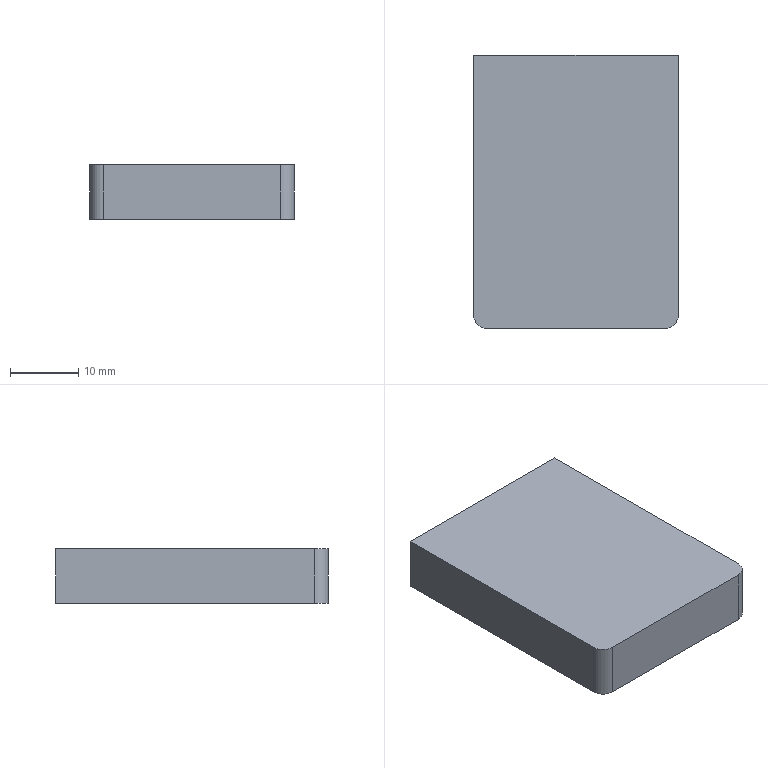Component | SolidWorks | GripperJaw2-1 | 1 solid | 8 faces | box 30 x 40 x 8 mm | volume 9586 mm3 | plane 6 | cylinder 2 | commonest cylinder face diameters 4 x2 | material 1060 Alloy
build123d program:
from build123d import *

# Parameters (mm, degrees)
SKETCH1_W           = 30
SKETCH1_H           = 40
BOSS_EXTRUDE1_DEPTH = 8
FILLET1_R           = 2


with BuildPart() as part:
    # Sketch1 → Boss-Extrude1 (new body)
    with BuildSketch(Plane.XY):
        Rectangle(SKETCH1_W, SKETCH1_H)
    extrude(amount=BOSS_EXTRUDE1_DEPTH)

    # Fillet1
    fillet1_edges = [part.edges().sort_by_distance(p)[0] for p in [
        (15, -20, 4),
        (-15, -20, 4),
    ]]
    fillet(fillet1_edges, radius=FILLET1_R)


solid = part.part

# Placed as in the assembly
solid = solid.moved(Location((-45.188, -89.343, 182.72), (0, 0, 0)))
STEP:
#1=COLOUR_RGB('',0.7922,0.8196,0.9333);
#2=FILL_AREA_STYLE_COLOUR('',#1);
#3=FILL_AREA_STYLE('',(#2));
#4=SURFACE_STYLE_FILL_AREA(#3);
#5=SURFACE_SIDE_STYLE('',(#4));
#6=SURFACE_STYLE_USAGE(.BOTH.,#5);
#7=PRESENTATION_STYLE_ASSIGNMENT((#6));
#8=CARTESIAN_POINT('',(-1.188,-4.226,7.509));
#9=VERTEX_POINT('',#8);
#10=CARTESIAN_POINT('',(-1.188,-2.73,7.509));
#11=VERTEX_POINT('',#10);
#12=CARTESIAN_POINT('',(-1.188,-2.73,7.509));
#13=DIRECTION('',(-0.,1.,0.));
#14=VECTOR('',#13,39.37);
#15=LINE('',#12,#14);
#16=EDGE_CURVE('',#9,#11,#15,.T.);
#17=ORIENTED_EDGE('',*,*,#16,.F.);
#18=CARTESIAN_POINT('',(-1.188,-4.226,7.194));
#19=VERTEX_POINT('',#18);
#20=CARTESIAN_POINT('',(-1.188,-4.226,7.509));
#21=DIRECTION('',(0.,0.,-1.));
#22=VECTOR('',#21,39.37);
#23=LINE('',#20,#22);
#24=EDGE_CURVE('',#9,#19,#23,.T.);
#25=ORIENTED_EDGE('',*,*,#24,.T.);
#26=CARTESIAN_POINT('',(-1.188,-2.73,7.194));
#27=VERTEX_POINT('',#26);
#28=CARTESIAN_POINT('',(-1.188,-2.73,7.194));
#29=DIRECTION('',(-0.,1.,0.));
#30=VECTOR('',#29,39.37);
#31=LINE('',#28,#30);
#32=EDGE_CURVE('',#19,#27,#31,.T.);
#33=ORIENTED_EDGE('',*,*,#32,.T.);
#34=CARTESIAN_POINT('',(-1.188,-2.73,7.509));
#35=DIRECTION('',(0.,0.,-1.));
#36=VECTOR('',#35,39.37);
#37=LINE('',#34,#36);
#38=EDGE_CURVE('',#11,#27,#37,.T.);
#39=ORIENTED_EDGE('',*,*,#38,.F.);
#40=EDGE_LOOP('',(#17,#25,#33,#39));
#41=FACE_OUTER_BOUND('',#40,.T.);
#42=CARTESIAN_POINT('',(-1.188,-2.73,7.509));
#43=DIRECTION('',(-1.,-0.,0.));
#44=DIRECTION('',(0.,-1.,0.));
#45=AXIS2_PLACEMENT_3D('',#42,#43,#44);
#46=PLANE('',#45);
#47=ADVANCED_FACE('',(#41),#46,.F.);
#48=CARTESIAN_POINT('',(-2.37,-2.73,7.194));
#49=VERTEX_POINT('',#48);
#50=CARTESIAN_POINT('',(-2.37,-2.73,7.194));
#51=DIRECTION('',(-1.,0.,0.));
#52=VECTOR('',#51,39.37);
#53=LINE('',#50,#52);
#54=EDGE_CURVE('',#27,#49,#53,.T.);
#55=ORIENTED_EDGE('',*,*,#54,.T.);
#56=CARTESIAN_POINT('',(-2.37,-2.73,7.509));
#57=VERTEX_POINT('',#56);
#58=CARTESIAN_POINT('',(-2.37,-2.73,7.509));
#59=DIRECTION('',(0.,0.,-1.));
#60=VECTOR('',#59,39.37);
#61=LINE('',#58,#60);
#62=EDGE_CURVE('',#57,#49,#61,.T.);
#63=ORIENTED_EDGE('',*,*,#62,.F.);
#64=CARTESIAN_POINT('',(-2.37,-2.73,7.509));
#65=DIRECTION('',(-1.,0.,0.));
#66=VECTOR('',#65,39.37);
#67=LINE('',#64,#66);
#68=EDGE_CURVE('',#11,#57,#67,.T.);
#69=ORIENTED_EDGE('',*,*,#68,.F.);
#70=ORIENTED_EDGE('',*,*,#38,.T.);
#71=EDGE_LOOP('',(#55,#63,#69,#70));
#72=FACE_OUTER_BOUND('',#71,.T.);
#73=CARTESIAN_POINT('',(-2.37,-2.73,7.509));
#74=DIRECTION('',(0.,-1.,0.));
#75=DIRECTION('',(0.,0.,-1.));
#76=AXIS2_PLACEMENT_3D('',#73,#74,#75);
#77=PLANE('',#76);
#78=ADVANCED_FACE('',(#72),#77,.F.);
#79=CARTESIAN_POINT('',(-2.37,-4.226,7.194));
#80=VERTEX_POINT('',#79);
#81=CARTESIAN_POINT('',(-2.37,-2.73,7.194));
#82=DIRECTION('',(0.,-1.,0.));
#83=VECTOR('',#82,39.37);
#84=LINE('',#81,#83);
#85=EDGE_CURVE('',#49,#80,#84,.T.);
#86=ORIENTED_EDGE('',*,*,#85,.T.);
#87=CARTESIAN_POINT('',(-2.37,-4.226,7.509));
#88=VERTEX_POINT('',#87);
#89=CARTESIAN_POINT('',(-2.37,-4.226,7.509));
#90=DIRECTION('',(0.,0.,1.));
#91=VECTOR('',#90,39.37);
#92=LINE('',#89,#91);
#93=EDGE_CURVE('',#80,#88,#92,.T.);
#94=ORIENTED_EDGE('',*,*,#93,.T.);
#95=CARTESIAN_POINT('',(-2.37,-2.73,7.509));
#96=DIRECTION('',(0.,-1.,0.));
#97=VECTOR('',#96,39.37);
#98=LINE('',#95,#97);
#99=EDGE_CURVE('',#57,#88,#98,.T.);
#100=ORIENTED_EDGE('',*,*,#99,.F.);
#101=ORIENTED_EDGE('',*,*,#62,.T.);
#102=EDGE_LOOP('',(#86,#94,#100,#101));
#103=FACE_OUTER_BOUND('',#102,.T.);
#104=CARTESIAN_POINT('',(-2.37,-2.73,7.509));
#105=DIRECTION('',(1.,0.,0.));
#106=DIRECTION('',(-0.,1.,0.));
#107=AXIS2_PLACEMENT_3D('',#104,#105,#106);
#108=PLANE('',#107);
#109=ADVANCED_FACE('',(#103),#108,.F.);
#110=CARTESIAN_POINT('',(-2.291,-4.305,7.194));
#111=VERTEX_POINT('',#110);
#112=CARTESIAN_POINT('',(-1.267,-4.305,7.194));
#113=VERTEX_POINT('',#112);
#114=CARTESIAN_POINT('',(-2.37,-4.305,7.194));
#115=DIRECTION('',(1.,0.,0.));
#116=VECTOR('',#115,39.37);
#117=LINE('',#114,#116);
#118=EDGE_CURVE('',#111,#113,#117,.T.);
#119=ORIENTED_EDGE('',*,*,#118,.T.);
#120=CARTESIAN_POINT('',(-1.267,-4.305,7.509));
#121=VERTEX_POINT('',#120);
#122=CARTESIAN_POINT('',(-1.267,-4.305,7.509));
#123=DIRECTION('',(0.,0.,1.));
#124=VECTOR('',#123,39.37);
#125=LINE('',#122,#124);
#126=EDGE_CURVE('',#113,#121,#125,.T.);
#127=ORIENTED_EDGE('',*,*,#126,.T.);
#128=CARTESIAN_POINT('',(-2.291,-4.305,7.509));
#129=VERTEX_POINT('',#128);
#130=CARTESIAN_POINT('',(-2.37,-4.305,7.509));
#131=DIRECTION('',(1.,0.,0.));
#132=VECTOR('',#131,39.37);
#133=LINE('',#130,#132);
#134=EDGE_CURVE('',#129,#121,#133,.T.);
#135=ORIENTED_EDGE('',*,*,#134,.F.);
#136=CARTESIAN_POINT('',(-2.291,-4.305,7.509));
#137=DIRECTION('',(0.,0.,-1.));
#138=VECTOR('',#137,39.37);
#139=LINE('',#136,#138);
#140=EDGE_CURVE('',#129,#111,#139,.T.);
#141=ORIENTED_EDGE('',*,*,#140,.T.);
#142=EDGE_LOOP('',(#119,#127,#135,#141));
#143=FACE_OUTER_BOUND('',#142,.T.);
#144=CARTESIAN_POINT('',(-2.37,-4.305,7.509));
#145=DIRECTION('',(0.,1.,0.));
#146=DIRECTION('',(0.,0.,1.));
#147=AXIS2_PLACEMENT_3D('',#144,#145,#146);
#148=PLANE('',#147);
#149=ADVANCED_FACE('',(#143),#148,.F.);
#150=ORIENTED_EDGE('',*,*,#134,.T.);
#151=CARTESIAN_POINT('',(-1.267,-4.226,7.509));
#152=DIRECTION('',(0.,0.,1.));
#153=DIRECTION('',(1.,0.,0.));
#154=AXIS2_PLACEMENT_3D('',#151,#152,#153);
#155=CIRCLE('',#154,0.07874);
#156=EDGE_CURVE('',#121,#9,#155,.T.);
#157=ORIENTED_EDGE('',*,*,#156,.T.);
#158=ORIENTED_EDGE('',*,*,#16,.T.);
#159=ORIENTED_EDGE('',*,*,#68,.T.);
#160=ORIENTED_EDGE('',*,*,#99,.T.);
#161=CARTESIAN_POINT('',(-2.291,-4.226,7.509));
#162=DIRECTION('',(0.,0.,1.));
#163=DIRECTION('',(1.,0.,0.));
#164=AXIS2_PLACEMENT_3D('',#161,#162,#163);
#165=CIRCLE('',#164,0.07874);
#166=EDGE_CURVE('',#88,#129,#165,.T.);
#167=ORIENTED_EDGE('',*,*,#166,.T.);
#168=EDGE_LOOP('',(#150,#157,#158,#159,#160,#167));
#169=FACE_OUTER_BOUND('',#168,.T.);
#170=CARTESIAN_POINT('',(-1.779,-3.517,7.509));
#171=DIRECTION('',(0.,0.,1.));
#172=DIRECTION('',(1.,0.,0.));
#173=AXIS2_PLACEMENT_3D('',#170,#171,#172);
#174=PLANE('',#173);
#175=ADVANCED_FACE('',(#169),#174,.T.);
#176=ORIENTED_EDGE('',*,*,#32,.F.);
#177=CARTESIAN_POINT('',(-1.267,-4.226,7.194));
#178=DIRECTION('',(0.,0.,-1.));
#179=DIRECTION('',(1.,0.,0.));
#180=AXIS2_PLACEMENT_3D('',#177,#178,#179);
#181=CIRCLE('',#180,0.07874);
#182=EDGE_CURVE('',#19,#113,#181,.T.);
#183=ORIENTED_EDGE('',*,*,#182,.T.);
#184=ORIENTED_EDGE('',*,*,#118,.F.);
#185=CARTESIAN_POINT('',(-2.291,-4.226,7.194));
#186=DIRECTION('',(0.,0.,-1.));
#187=DIRECTION('',(1.,0.,0.));
#188=AXIS2_PLACEMENT_3D('',#185,#186,#187);
#189=CIRCLE('',#188,0.07874);
#190=EDGE_CURVE('',#111,#80,#189,.T.);
#191=ORIENTED_EDGE('',*,*,#190,.T.);
#192=ORIENTED_EDGE('',*,*,#85,.F.);
#193=ORIENTED_EDGE('',*,*,#54,.F.);
#194=EDGE_LOOP('',(#176,#183,#184,#191,#192,#193));
#195=FACE_OUTER_BOUND('',#194,.T.);
#196=CARTESIAN_POINT('',(-1.779,-3.517,7.194));
#197=DIRECTION('',(0.,0.,1.));
#198=DIRECTION('',(1.,0.,0.));
#199=AXIS2_PLACEMENT_3D('',#196,#197,#198);
#200=PLANE('',#199);
#201=ADVANCED_FACE('',(#195),#200,.F.);
#202=ORIENTED_EDGE('',*,*,#156,.F.);
#203=ORIENTED_EDGE('',*,*,#126,.F.);
#204=ORIENTED_EDGE('',*,*,#182,.F.);
#205=ORIENTED_EDGE('',*,*,#24,.F.);
#206=EDGE_LOOP('',(#202,#203,#204,#205));
#207=FACE_OUTER_BOUND('',#206,.T.);
#208=CARTESIAN_POINT('',(-1.267,-4.226,7.509));
#209=DIRECTION('',(0.,0.,-1.));
#210=DIRECTION('',(-1.,0.,0.));
#211=AXIS2_PLACEMENT_3D('',#208,#209,#210);
#212=CYLINDRICAL_SURFACE('',#211,0.07874);
#213=ADVANCED_FACE('',(#207),#212,.T.);
#214=ORIENTED_EDGE('',*,*,#166,.F.);
#215=ORIENTED_EDGE('',*,*,#93,.F.);
#216=ORIENTED_EDGE('',*,*,#190,.F.);
#217=ORIENTED_EDGE('',*,*,#140,.F.);
#218=EDGE_LOOP('',(#214,#215,#216,#217));
#219=FACE_OUTER_BOUND('',#218,.T.);
#220=CARTESIAN_POINT('',(-2.291,-4.226,7.509));
#221=DIRECTION('',(0.,0.,-1.));
#222=DIRECTION('',(-1.,0.,0.));
#223=AXIS2_PLACEMENT_3D('',#220,#221,#222);
#224=CYLINDRICAL_SURFACE('',#223,0.07874);
#225=ADVANCED_FACE('',(#219),#224,.T.);
#226=CLOSED_SHELL('',(#47,#78,#109,#149,#175,#201,#213,#225));
#227=MANIFOLD_SOLID_BREP('',#226);
#228=STYLED_ITEM('',(#7),#227);
#229=PRESENTATION_LAYER_ASSIGNMENT('','',(#228));
#230=CARTESIAN_POINT('',(0.,0.,0.));
#231=DIRECTION('',(0.,0.,1.));
#232=DIRECTION('',(1.,0.,0.));
#233=AXIS2_PLACEMENT_3D('',#230,#231,#232);
#234=(LENGTH_UNIT()NAMED_UNIT(*)SI_UNIT($,.METRE.));
#235=LENGTH_MEASURE_WITH_UNIT(LENGTH_MEASURE(0.0254),#234);
#236=DIMENSIONAL_EXPONENTS(1.,0.,0.,0.,0.,0.,0.);
#237=(CONVERSION_BASED_UNIT('',#235)LENGTH_UNIT()NAMED_UNIT(#236));
#238=UNCERTAINTY_MEASURE_WITH_UNIT(LENGTH_MEASURE(0.00001),#237,'','');
#239=(NAMED_UNIT(*)PLANE_ANGLE_UNIT()SI_UNIT($,.RADIAN.));
#240=(NAMED_UNIT(*)SI_UNIT($,.STERADIAN.)SOLID_ANGLE_UNIT());
#241=(GEOMETRIC_REPRESENTATION_CONTEXT(3)GLOBAL_UNCERTAINTY_ASSIGNED_CONTEXT((#238))GLOBAL_UNIT_ASSIGNED_CONTEXT((#237,#239,#240))REPRESENTATION_CONTEXT('',''));
#242=ADVANCED_BREP_SHAPE_REPRESENTATION('',(#227,#233),#241);
#243=(LENGTH_UNIT()NAMED_UNIT(*)SI_UNIT($,.METRE.));
#244=LENGTH_MEASURE_WITH_UNIT(LENGTH_MEASURE(0.0254),#243);
#245=DIMENSIONAL_EXPONENTS(1.,0.,0.,0.,0.,0.,0.);
#246=(CONVERSION_BASED_UNIT('',#244)LENGTH_UNIT()NAMED_UNIT(#245));
#247=UNCERTAINTY_MEASURE_WITH_UNIT(LENGTH_MEASURE(0.00001),#246,'','');
#248=(NAMED_UNIT(*)PLANE_ANGLE_UNIT()SI_UNIT($,.RADIAN.));
#249=(NAMED_UNIT(*)SI_UNIT($,.STERADIAN.)SOLID_ANGLE_UNIT());
#250=(GEOMETRIC_REPRESENTATION_CONTEXT(3)GLOBAL_UNCERTAINTY_ASSIGNED_CONTEXT((#247))GLOBAL_UNIT_ASSIGNED_CONTEXT((#246,#248,#249))REPRESENTATION_CONTEXT('',''));
#251=MECHANICAL_DESIGN_GEOMETRIC_PRESENTATION_REPRESENTATION('',(#228),#250);